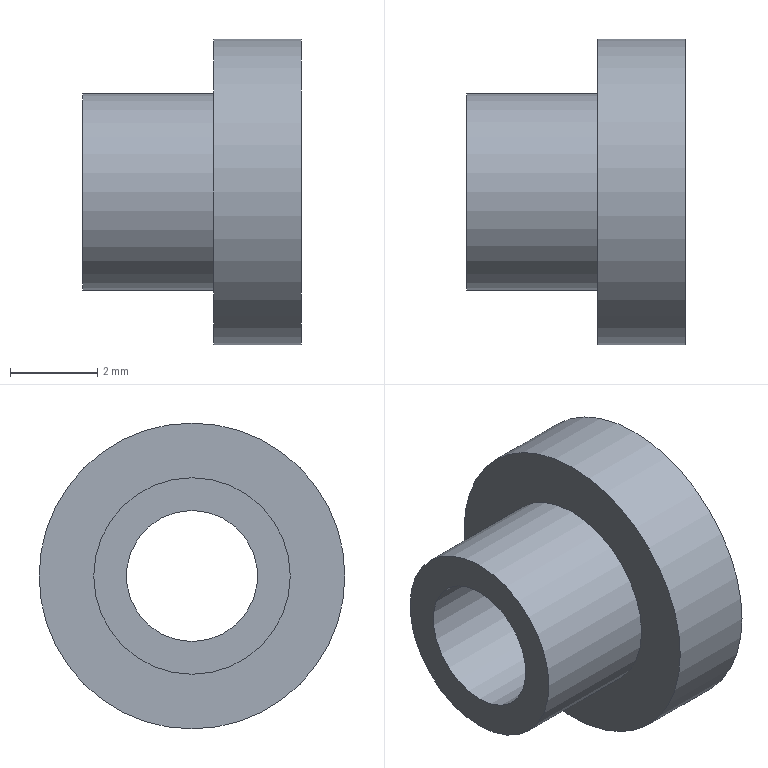Component | NX | EXT_CYLINDER_BODY_SHAFT_SLEEVE | 1 solid | 6 faces | volume 89 mm3 | plane 3 | cylinder 3 | commonest cylinder face diameters 4.5 x1 7 x1 3 x1